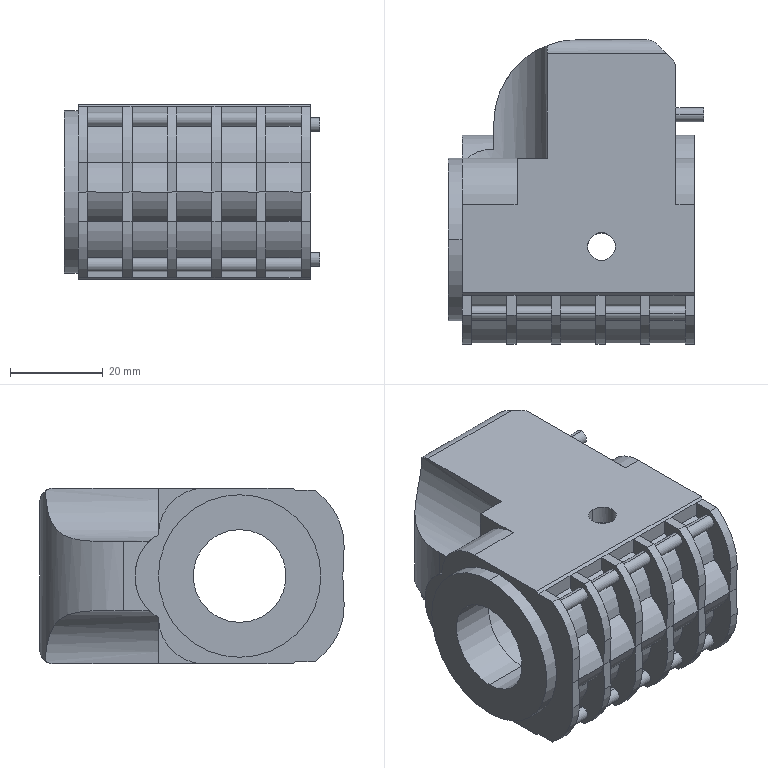Component | SolidWorks | 3-1 | 1 solid | 159 faces | volume 67131 mm3 | cylinder 84 | plane 75 | commonest cylinder face diameters 20 x30 3 x24 30 x14 6 x8 23 x3 2 x2 35 x2 36 x1